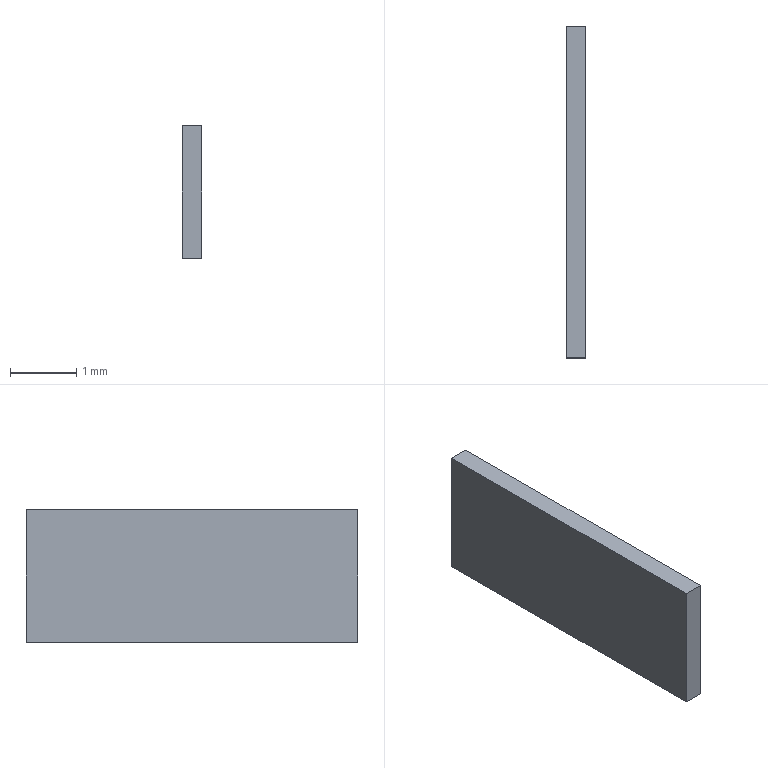Component | NX | SENSOR_43_2 | 1 solid | 6 faces | box 0.3 x 5 x 2 mm | volume 3 mm3 | plane 6
STEP:
#1=CARTESIAN_POINT('',(0.,0.,0.));
#2=DIRECTION('',(0.,0.,1.));
#3=DIRECTION('',(1.,0.,0.));
#4=AXIS2_PLACEMENT_3D('',#1,#2,#3);
#5=CARTESIAN_POINT('',(-93.731,18.5,14.));
#6=VERTEX_POINT('',#5);
#7=CARTESIAN_POINT('',(-93.731,13.5,14.));
#8=VERTEX_POINT('',#7);
#9=CARTESIAN_POINT('',(-93.731,16.,14.));
#10=DIRECTION('',(0.,-1.,0.));
#11=VECTOR('',#10,1.);
#12=LINE('',#9,#11);
#13=CARTESIAN_POINT('',(-93.881,16.,14.));
#14=DIRECTION('',(0.,0.,1.));
#15=DIRECTION('',(0.,1.,0.));
#16=AXIS2_PLACEMENT_3D('',#13,#14,#15);
#17=PLANE('',#16);
#18=CARTESIAN_POINT('',(0.,-0.15));
#19=DIRECTION('',(-1.,0.));
#20=VECTOR('',#19,1.);
#21=LINE('',#18,#20);
#22=(GEOMETRIC_REPRESENTATION_CONTEXT(2)PARAMETRIC_REPRESENTATION_CONTEXT()REPRESENTATION_CONTEXT('',''));
#23=DEFINITIONAL_REPRESENTATION('',(#21),#22);
#24=PCURVE('',#17,#23);
#25=CARTESIAN_POINT('',(-93.731,16.,12.));
#26=DIRECTION('',(1.,0.,0.));
#27=DIRECTION('',(0.,0.,-1.));
#28=AXIS2_PLACEMENT_3D('',#25,#26,#27);
#29=PLANE('',#28);
#30=CARTESIAN_POINT('',(-2.,0.));
#31=DIRECTION('',(0.,-1.));
#32=VECTOR('',#31,1.);
#33=LINE('',#30,#32);
#34=(GEOMETRIC_REPRESENTATION_CONTEXT(2)PARAMETRIC_REPRESENTATION_CONTEXT()REPRESENTATION_CONTEXT('',''));
#35=DEFINITIONAL_REPRESENTATION('',(#33),#34);
#36=PCURVE('',#29,#35);
#37=SURFACE_CURVE('',#12,(#24,#36),.PCURVE_S1.);
#38=EDGE_CURVE('',#6,#8,#37,.T.);
#39=ORIENTED_EDGE('',*,*,#38,.F.);
#40=CARTESIAN_POINT('',(-94.031,18.5,14.));
#41=VERTEX_POINT('',#40);
#42=CARTESIAN_POINT('',(-93.881,18.5,14.));
#43=DIRECTION('',(1.,0.,0.));
#44=VECTOR('',#43,1.);
#45=LINE('',#42,#44);
#46=CARTESIAN_POINT('',(2.5,0.));
#47=DIRECTION('',(0.,-1.));
#48=VECTOR('',#47,1.);
#49=LINE('',#46,#48);
#50=(GEOMETRIC_REPRESENTATION_CONTEXT(2)PARAMETRIC_REPRESENTATION_CONTEXT()REPRESENTATION_CONTEXT('',''));
#51=DEFINITIONAL_REPRESENTATION('',(#49),#50);
#52=PCURVE('',#17,#51);
#53=CARTESIAN_POINT('',(-93.881,18.5,12.));
#54=DIRECTION('',(0.,1.,0.));
#55=DIRECTION('',(0.,0.,-1.));
#56=AXIS2_PLACEMENT_3D('',#53,#54,#55);
#57=PLANE('',#56);
#58=CARTESIAN_POINT('',(-2.,0.));
#59=DIRECTION('',(0.,-1.));
#60=VECTOR('',#59,1.);
#61=LINE('',#58,#60);
#62=(GEOMETRIC_REPRESENTATION_CONTEXT(2)PARAMETRIC_REPRESENTATION_CONTEXT()REPRESENTATION_CONTEXT('',''));
#63=DEFINITIONAL_REPRESENTATION('',(#61),#62);
#64=PCURVE('',#57,#63);
#65=SURFACE_CURVE('',#45,(#52,#64),.PCURVE_S1.);
#66=EDGE_CURVE('',#41,#6,#65,.T.);
#67=ORIENTED_EDGE('',*,*,#66,.F.);
#68=CARTESIAN_POINT('',(-94.031,13.5,14.));
#69=VERTEX_POINT('',#68);
#70=CARTESIAN_POINT('',(-94.031,16.,14.));
#71=DIRECTION('',(0.,1.,0.));
#72=VECTOR('',#71,1.);
#73=LINE('',#70,#72);
#74=CARTESIAN_POINT('',(0.,0.15));
#75=DIRECTION('',(1.,0.));
#76=VECTOR('',#75,1.);
#77=LINE('',#74,#76);
#78=(GEOMETRIC_REPRESENTATION_CONTEXT(2)PARAMETRIC_REPRESENTATION_CONTEXT()REPRESENTATION_CONTEXT('',''));
#79=DEFINITIONAL_REPRESENTATION('',(#77),#78);
#80=PCURVE('',#17,#79);
#81=CARTESIAN_POINT('',(-94.031,16.,12.));
#82=DIRECTION('',(-1.,0.,0.));
#83=DIRECTION('',(0.,0.,1.));
#84=AXIS2_PLACEMENT_3D('',#81,#82,#83);
#85=PLANE('',#84);
#86=CARTESIAN_POINT('',(2.,0.));
#87=DIRECTION('',(0.,1.));
#88=VECTOR('',#87,1.);
#89=LINE('',#86,#88);
#90=(GEOMETRIC_REPRESENTATION_CONTEXT(2)PARAMETRIC_REPRESENTATION_CONTEXT()REPRESENTATION_CONTEXT('',''));
#91=DEFINITIONAL_REPRESENTATION('',(#89),#90);
#92=PCURVE('',#85,#91);
#93=SURFACE_CURVE('',#73,(#80,#92),.PCURVE_S1.);
#94=EDGE_CURVE('',#69,#41,#93,.T.);
#95=ORIENTED_EDGE('',*,*,#94,.F.);
#96=CARTESIAN_POINT('',(-93.881,13.5,14.));
#97=DIRECTION('',(-1.,0.,0.));
#98=VECTOR('',#97,1.);
#99=LINE('',#96,#98);
#100=CARTESIAN_POINT('',(-2.5,0.));
#101=DIRECTION('',(0.,1.));
#102=VECTOR('',#101,1.);
#103=LINE('',#100,#102);
#104=(GEOMETRIC_REPRESENTATION_CONTEXT(2)PARAMETRIC_REPRESENTATION_CONTEXT()REPRESENTATION_CONTEXT('',''));
#105=DEFINITIONAL_REPRESENTATION('',(#103),#104);
#106=PCURVE('',#17,#105);
#107=CARTESIAN_POINT('',(-93.881,13.5,12.));
#108=DIRECTION('',(0.,-1.,0.));
#109=DIRECTION('',(0.,0.,1.));
#110=AXIS2_PLACEMENT_3D('',#107,#108,#109);
#111=PLANE('',#110);
#112=CARTESIAN_POINT('',(2.,0.));
#113=DIRECTION('',(0.,1.));
#114=VECTOR('',#113,1.);
#115=LINE('',#112,#114);
#116=(GEOMETRIC_REPRESENTATION_CONTEXT(2)PARAMETRIC_REPRESENTATION_CONTEXT()REPRESENTATION_CONTEXT('',''));
#117=DEFINITIONAL_REPRESENTATION('',(#115),#116);
#118=PCURVE('',#111,#117);
#119=SURFACE_CURVE('',#99,(#106,#118),.PCURVE_S1.);
#120=EDGE_CURVE('',#8,#69,#119,.T.);
#121=ORIENTED_EDGE('',*,*,#120,.F.);
#122=EDGE_LOOP('',(#39,#67,#95,#121));
#123=FACE_BOUND('',#122,.T.);
#124=ADVANCED_FACE('',(#123),#17,.T.);
#125=CARTESIAN_POINT('',(-93.731,18.5,12.));
#126=VERTEX_POINT('',#125);
#127=CARTESIAN_POINT('',(-93.731,18.5,12.));
#128=DIRECTION('',(0.,0.,1.));
#129=VECTOR('',#128,1.);
#130=LINE('',#127,#129);
#131=CARTESIAN_POINT('',(0.,2.5));
#132=DIRECTION('',(-1.,0.));
#133=VECTOR('',#132,1.);
#134=LINE('',#131,#133);
#135=(GEOMETRIC_REPRESENTATION_CONTEXT(2)PARAMETRIC_REPRESENTATION_CONTEXT()REPRESENTATION_CONTEXT('',''));
#136=DEFINITIONAL_REPRESENTATION('',(#134),#135);
#137=PCURVE('',#29,#136);
#138=CARTESIAN_POINT('',(0.,-0.15));
#139=DIRECTION('',(-1.,0.));
#140=VECTOR('',#139,1.);
#141=LINE('',#138,#140);
#142=(GEOMETRIC_REPRESENTATION_CONTEXT(2)PARAMETRIC_REPRESENTATION_CONTEXT()REPRESENTATION_CONTEXT('',''));
#143=DEFINITIONAL_REPRESENTATION('',(#141),#142);
#144=PCURVE('',#57,#143);
#145=SURFACE_CURVE('',#130,(#137,#144),.PCURVE_S1.);
#146=EDGE_CURVE('',#126,#6,#145,.T.);
#147=ORIENTED_EDGE('',*,*,#146,.T.);
#148=ORIENTED_EDGE('',*,*,#38,.T.);
#149=CARTESIAN_POINT('',(-93.731,13.5,12.));
#150=VERTEX_POINT('',#149);
#151=CARTESIAN_POINT('',(-93.731,13.5,12.));
#152=DIRECTION('',(0.,0.,1.));
#153=VECTOR('',#152,1.);
#154=LINE('',#151,#153);
#155=CARTESIAN_POINT('',(0.,-2.5));
#156=DIRECTION('',(-1.,0.));
#157=VECTOR('',#156,1.);
#158=LINE('',#155,#157);
#159=(GEOMETRIC_REPRESENTATION_CONTEXT(2)PARAMETRIC_REPRESENTATION_CONTEXT()REPRESENTATION_CONTEXT('',''));
#160=DEFINITIONAL_REPRESENTATION('',(#158),#159);
#161=PCURVE('',#29,#160);
#162=CARTESIAN_POINT('',(0.,-0.15));
#163=DIRECTION('',(1.,0.));
#164=VECTOR('',#163,1.);
#165=LINE('',#162,#164);
#166=(GEOMETRIC_REPRESENTATION_CONTEXT(2)PARAMETRIC_REPRESENTATION_CONTEXT()REPRESENTATION_CONTEXT('',''));
#167=DEFINITIONAL_REPRESENTATION('',(#165),#166);
#168=PCURVE('',#111,#167);
#169=SURFACE_CURVE('',#154,(#161,#168),.PCURVE_S1.);
#170=EDGE_CURVE('',#150,#8,#169,.T.);
#171=ORIENTED_EDGE('',*,*,#170,.F.);
#172=CARTESIAN_POINT('',(-93.731,16.,12.));
#173=DIRECTION('',(0.,1.,0.));
#174=VECTOR('',#173,1.);
#175=LINE('',#172,#174);
#176=CARTESIAN_POINT('',(0.,0.));
#177=DIRECTION('',(0.,1.));
#178=VECTOR('',#177,1.);
#179=LINE('',#176,#178);
#180=(GEOMETRIC_REPRESENTATION_CONTEXT(2)PARAMETRIC_REPRESENTATION_CONTEXT()REPRESENTATION_CONTEXT('',''));
#181=DEFINITIONAL_REPRESENTATION('',(#179),#180);
#182=PCURVE('',#29,#181);
#183=CARTESIAN_POINT('',(-93.881,16.,12.));
#184=DIRECTION('',(0.,0.,-1.));
#185=DIRECTION('',(0.,-1.,0.));
#186=AXIS2_PLACEMENT_3D('',#183,#184,#185);
#187=PLANE('',#186);
#188=CARTESIAN_POINT('',(0.,-0.15));
#189=DIRECTION('',(-1.,0.));
#190=VECTOR('',#189,1.);
#191=LINE('',#188,#190);
#192=(GEOMETRIC_REPRESENTATION_CONTEXT(2)PARAMETRIC_REPRESENTATION_CONTEXT()REPRESENTATION_CONTEXT('',''));
#193=DEFINITIONAL_REPRESENTATION('',(#191),#192);
#194=PCURVE('',#187,#193);
#195=SURFACE_CURVE('',#175,(#182,#194),.PCURVE_S1.);
#196=EDGE_CURVE('',#150,#126,#195,.T.);
#197=ORIENTED_EDGE('',*,*,#196,.T.);
#198=EDGE_LOOP('',(#147,#148,#171,#197));
#199=FACE_BOUND('',#198,.T.);
#200=ADVANCED_FACE('',(#199),#29,.T.);
#201=ORIENTED_EDGE('',*,*,#170,.T.);
#202=ORIENTED_EDGE('',*,*,#120,.T.);
#203=CARTESIAN_POINT('',(-94.031,13.5,12.));
#204=VERTEX_POINT('',#203);
#205=CARTESIAN_POINT('',(-94.031,13.5,12.));
#206=DIRECTION('',(0.,0.,1.));
#207=VECTOR('',#206,1.);
#208=LINE('',#205,#207);
#209=CARTESIAN_POINT('',(0.,0.15));
#210=DIRECTION('',(1.,0.));
#211=VECTOR('',#210,1.);
#212=LINE('',#209,#211);
#213=(GEOMETRIC_REPRESENTATION_CONTEXT(2)PARAMETRIC_REPRESENTATION_CONTEXT()REPRESENTATION_CONTEXT('',''));
#214=DEFINITIONAL_REPRESENTATION('',(#212),#213);
#215=PCURVE('',#111,#214);
#216=CARTESIAN_POINT('',(0.,-2.5));
#217=DIRECTION('',(1.,0.));
#218=VECTOR('',#217,1.);
#219=LINE('',#216,#218);
#220=(GEOMETRIC_REPRESENTATION_CONTEXT(2)PARAMETRIC_REPRESENTATION_CONTEXT()REPRESENTATION_CONTEXT('',''));
#221=DEFINITIONAL_REPRESENTATION('',(#219),#220);
#222=PCURVE('',#85,#221);
#223=SURFACE_CURVE('',#208,(#215,#222),.PCURVE_S1.);
#224=EDGE_CURVE('',#204,#69,#223,.T.);
#225=ORIENTED_EDGE('',*,*,#224,.F.);
#226=CARTESIAN_POINT('',(-93.881,13.5,12.));
#227=DIRECTION('',(1.,0.,0.));
#228=VECTOR('',#227,1.);
#229=LINE('',#226,#228);
#230=CARTESIAN_POINT('',(0.,0.));
#231=DIRECTION('',(0.,-1.));
#232=VECTOR('',#231,1.);
#233=LINE('',#230,#232);
#234=(GEOMETRIC_REPRESENTATION_CONTEXT(2)PARAMETRIC_REPRESENTATION_CONTEXT()REPRESENTATION_CONTEXT('',''));
#235=DEFINITIONAL_REPRESENTATION('',(#233),#234);
#236=PCURVE('',#111,#235);
#237=CARTESIAN_POINT('',(2.5,0.));
#238=DIRECTION('',(0.,-1.));
#239=VECTOR('',#238,1.);
#240=LINE('',#237,#239);
#241=(GEOMETRIC_REPRESENTATION_CONTEXT(2)PARAMETRIC_REPRESENTATION_CONTEXT()REPRESENTATION_CONTEXT('',''));
#242=DEFINITIONAL_REPRESENTATION('',(#240),#241);
#243=PCURVE('',#187,#242);
#244=SURFACE_CURVE('',#229,(#236,#243),.PCURVE_S1.);
#245=EDGE_CURVE('',#204,#150,#244,.T.);
#246=ORIENTED_EDGE('',*,*,#245,.T.);
#247=EDGE_LOOP('',(#201,#202,#225,#246));
#248=FACE_BOUND('',#247,.T.);
#249=ADVANCED_FACE('',(#248),#111,.T.);
#250=ORIENTED_EDGE('',*,*,#224,.T.);
#251=ORIENTED_EDGE('',*,*,#94,.T.);
#252=CARTESIAN_POINT('',(-94.031,18.5,12.));
#253=VERTEX_POINT('',#252);
#254=CARTESIAN_POINT('',(-94.031,18.5,12.));
#255=DIRECTION('',(0.,0.,1.));
#256=VECTOR('',#255,1.);
#257=LINE('',#254,#256);
#258=CARTESIAN_POINT('',(0.,2.5));
#259=DIRECTION('',(1.,0.));
#260=VECTOR('',#259,1.);
#261=LINE('',#258,#260);
#262=(GEOMETRIC_REPRESENTATION_CONTEXT(2)PARAMETRIC_REPRESENTATION_CONTEXT()REPRESENTATION_CONTEXT('',''));
#263=DEFINITIONAL_REPRESENTATION('',(#261),#262);
#264=PCURVE('',#85,#263);
#265=CARTESIAN_POINT('',(0.,0.15));
#266=DIRECTION('',(-1.,0.));
#267=VECTOR('',#266,1.);
#268=LINE('',#265,#267);
#269=(GEOMETRIC_REPRESENTATION_CONTEXT(2)PARAMETRIC_REPRESENTATION_CONTEXT()REPRESENTATION_CONTEXT('',''));
#270=DEFINITIONAL_REPRESENTATION('',(#268),#269);
#271=PCURVE('',#57,#270);
#272=SURFACE_CURVE('',#257,(#264,#271),.PCURVE_S1.);
#273=EDGE_CURVE('',#253,#41,#272,.T.);
#274=ORIENTED_EDGE('',*,*,#273,.F.);
#275=CARTESIAN_POINT('',(-94.031,16.,12.));
#276=DIRECTION('',(0.,-1.,0.));
#277=VECTOR('',#276,1.);
#278=LINE('',#275,#277);
#279=CARTESIAN_POINT('',(0.,0.));
#280=DIRECTION('',(0.,-1.));
#281=VECTOR('',#280,1.);
#282=LINE('',#279,#281);
#283=(GEOMETRIC_REPRESENTATION_CONTEXT(2)PARAMETRIC_REPRESENTATION_CONTEXT()REPRESENTATION_CONTEXT('',''));
#284=DEFINITIONAL_REPRESENTATION('',(#282),#283);
#285=PCURVE('',#85,#284);
#286=CARTESIAN_POINT('',(0.,0.15));
#287=DIRECTION('',(1.,0.));
#288=VECTOR('',#287,1.);
#289=LINE('',#286,#288);
#290=(GEOMETRIC_REPRESENTATION_CONTEXT(2)PARAMETRIC_REPRESENTATION_CONTEXT()REPRESENTATION_CONTEXT('',''));
#291=DEFINITIONAL_REPRESENTATION('',(#289),#290);
#292=PCURVE('',#187,#291);
#293=SURFACE_CURVE('',#278,(#285,#292),.PCURVE_S1.);
#294=EDGE_CURVE('',#253,#204,#293,.T.);
#295=ORIENTED_EDGE('',*,*,#294,.T.);
#296=EDGE_LOOP('',(#250,#251,#274,#295));
#297=FACE_BOUND('',#296,.T.);
#298=ADVANCED_FACE('',(#297),#85,.T.);
#299=CARTESIAN_POINT('',(-93.881,18.5,12.));
#300=DIRECTION('',(-1.,0.,0.));
#301=VECTOR('',#300,1.);
#302=LINE('',#299,#301);
#303=CARTESIAN_POINT('',(-2.5,0.));
#304=DIRECTION('',(0.,1.));
#305=VECTOR('',#304,1.);
#306=LINE('',#303,#305);
#307=(GEOMETRIC_REPRESENTATION_CONTEXT(2)PARAMETRIC_REPRESENTATION_CONTEXT()REPRESENTATION_CONTEXT('',''));
#308=DEFINITIONAL_REPRESENTATION('',(#306),#307);
#309=PCURVE('',#187,#308);
#310=CARTESIAN_POINT('',(0.,0.));
#311=DIRECTION('',(0.,1.));
#312=VECTOR('',#311,1.);
#313=LINE('',#310,#312);
#314=(GEOMETRIC_REPRESENTATION_CONTEXT(2)PARAMETRIC_REPRESENTATION_CONTEXT()REPRESENTATION_CONTEXT('',''));
#315=DEFINITIONAL_REPRESENTATION('',(#313),#314);
#316=PCURVE('',#57,#315);
#317=SURFACE_CURVE('',#302,(#309,#316),.PCURVE_S1.);
#318=EDGE_CURVE('',#126,#253,#317,.T.);
#319=ORIENTED_EDGE('',*,*,#318,.F.);
#320=ORIENTED_EDGE('',*,*,#196,.F.);
#321=ORIENTED_EDGE('',*,*,#245,.F.);
#322=ORIENTED_EDGE('',*,*,#294,.F.);
#323=EDGE_LOOP('',(#319,#320,#321,#322));
#324=FACE_BOUND('',#323,.T.);
#325=ADVANCED_FACE('',(#324),#187,.T.);
#326=ORIENTED_EDGE('',*,*,#318,.T.);
#327=ORIENTED_EDGE('',*,*,#273,.T.);
#328=ORIENTED_EDGE('',*,*,#66,.T.);
#329=ORIENTED_EDGE('',*,*,#146,.F.);
#330=EDGE_LOOP('',(#326,#327,#328,#329));
#331=FACE_BOUND('',#330,.T.);
#332=ADVANCED_FACE('',(#331),#57,.T.);
#333=CLOSED_SHELL('',(#124,#200,#249,#298,#325,#332));
#334=MANIFOLD_SOLID_BREP('',#333);
#335=(LENGTH_UNIT()NAMED_UNIT(*)SI_UNIT(.MILLI.,.METRE.));
#336=UNCERTAINTY_MEASURE_WITH_UNIT(LENGTH_MEASURE(0.0000001),#335,'','');
#337=(NAMED_UNIT(*)PLANE_ANGLE_UNIT()SI_UNIT($,.RADIAN.));
#338=(NAMED_UNIT(*)SI_UNIT($,.STERADIAN.)SOLID_ANGLE_UNIT());
#339=(GEOMETRIC_REPRESENTATION_CONTEXT(3)GLOBAL_UNCERTAINTY_ASSIGNED_CONTEXT((#336))GLOBAL_UNIT_ASSIGNED_CONTEXT((#335,#337,#338))REPRESENTATION_CONTEXT('',''));
#340=ADVANCED_BREP_SHAPE_REPRESENTATION('',(#4,#334),#339);